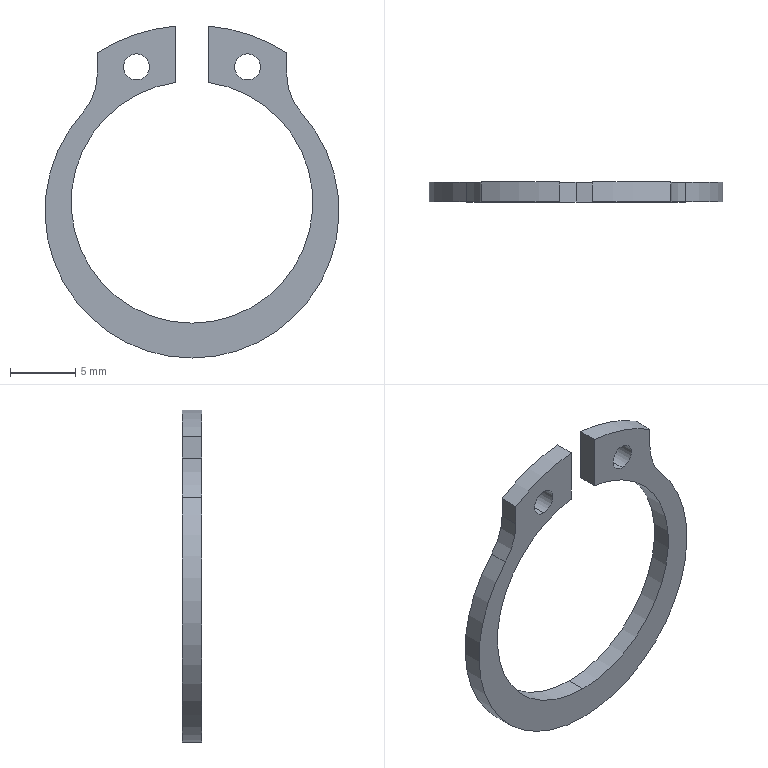Component | SolidWorks | 12-1 | 1 solid | 18 faces | box 22.5 x 1.5 x 25.41 mm | volume 237 mm3 | cylinder 12 | plane 6 | commonest cylinder face diameters 2 x4 18.5 x2 22.5 x2 27.1 x2 9 x2
build123d program:
from build123d import *

# Parameters (mm, degrees)
SKETCH1_R           = 1
BOSS_EXTRUDE1_DEPTH = 1.5
FILLET1_R           = 4.5


with BuildPart() as part:
    # Sketch1 → Boss-Extrude1 (new body)
    with BuildSketch(Plane(origin=(0, 0, 0), x_dir=(1, 0, 0), z_dir=(0, 1, 0))):
        with BuildLine():
            Line((7.25, -11.447), (7.25, -7.932))
            ThreePointArc((7.25, -7.932), (0, 11.92), (-7.25, -7.932))
            Line((-7.25, -7.932), (-7.25, -11.447))
            ThreePointArc((-7.25, -11.447), (-4.371, -12.826), (-1.25, -13.492))
            Line((-1.25, -13.492), (-1.25, -9.165))
            ThreePointArc((-1.25, -9.165), (0, 9.25), (1.25, -9.165))
            Line((1.25, -9.165), (1.25, -13.492))
            ThreePointArc((1.25, -13.492), (4.371, -12.826), (7.25, -11.447))
        make_face()
        with Locations(Location((-4.25, -10.362, 0), (0, 0, 270))):
            Circle(SKETCH1_R, mode=Mode.SUBTRACT)
        with Locations(Location((4.25, -10.362, 0), (0, 0, 90))):
            Circle(SKETCH1_R, mode=Mode.SUBTRACT)
    extrude(amount=BOSS_EXTRUDE1_DEPTH)

    # Fillet1
    fillet1_edges = [part.edges().sort_by_distance(p)[0] for p in [
        (7.25, 0.75, 7.932),
        (-7.25, 0.75, 7.932),
    ]]
    fillet(fillet1_edges, radius=FILLET1_R)


solid = part.part

# Placed as in the assembly
solid = solid.moved(Location((0, -59.437, 0), (0, 0, 0)))
STEP:
#1=COLOUR_RGB('',0.7922,0.8196,0.9333);
#2=FILL_AREA_STYLE_COLOUR('',#1);
#3=FILL_AREA_STYLE('',(#2));
#4=SURFACE_STYLE_FILL_AREA(#3);
#5=SURFACE_SIDE_STYLE('',(#4));
#6=SURFACE_STYLE_USAGE(.BOTH.,#5);
#7=PRESENTATION_STYLE_ASSIGNMENT((#6));
#8=CARTESIAN_POINT('',(0.1673,-2.281,0.3686));
#9=VERTEX_POINT('',#8);
#10=CARTESIAN_POINT('',(0.1673,-2.281,0.4473));
#11=VERTEX_POINT('',#10);
#12=CARTESIAN_POINT('',(0.1673,-2.281,0.408));
#13=DIRECTION('',(0.,1.,0.));
#14=DIRECTION('',(0.,0.,-1.));
#15=AXIS2_PLACEMENT_3D('',#12,#13,#14);
#16=CIRCLE('',#15,0.03937);
#17=EDGE_CURVE('',#9,#11,#16,.T.);
#18=ORIENTED_EDGE('',*,*,#17,.T.);
#19=CARTESIAN_POINT('',(0.1673,-2.34,0.4473));
#20=VERTEX_POINT('',#19);
#21=CARTESIAN_POINT('',(0.1673,-2.281,0.4473));
#22=DIRECTION('',(0.,-1.,0.));
#23=VECTOR('',#22,39.37);
#24=LINE('',#21,#23);
#25=EDGE_CURVE('',#11,#20,#24,.T.);
#26=ORIENTED_EDGE('',*,*,#25,.T.);
#27=CARTESIAN_POINT('',(0.1673,-2.34,0.3686));
#28=VERTEX_POINT('',#27);
#29=CARTESIAN_POINT('',(0.1673,-2.34,0.408));
#30=DIRECTION('',(0.,1.,0.));
#31=DIRECTION('',(0.,0.,-1.));
#32=AXIS2_PLACEMENT_3D('',#29,#30,#31);
#33=CIRCLE('',#32,0.03937);
#34=EDGE_CURVE('',#28,#20,#33,.T.);
#35=ORIENTED_EDGE('',*,*,#34,.F.);
#36=CARTESIAN_POINT('',(0.1673,-2.281,0.3686));
#37=DIRECTION('',(0.,-1.,0.));
#38=VECTOR('',#37,39.37);
#39=LINE('',#36,#38);
#40=EDGE_CURVE('',#9,#28,#39,.T.);
#41=ORIENTED_EDGE('',*,*,#40,.F.);
#42=EDGE_LOOP('',(#18,#26,#35,#41));
#43=FACE_OUTER_BOUND('',#42,.T.);
#44=CARTESIAN_POINT('',(0.1673,-2.281,0.408));
#45=DIRECTION('',(0.,-1.,0.));
#46=DIRECTION('',(0.,0.,-1.));
#47=AXIS2_PLACEMENT_3D('',#44,#45,#46);
#48=CYLINDRICAL_SURFACE('',#47,0.03937);
#49=ADVANCED_FACE('',(#43),#48,.F.);
#50=CARTESIAN_POINT('',(-0.1673,-2.281,0.3686));
#51=VERTEX_POINT('',#50);
#52=CARTESIAN_POINT('',(-0.1673,-2.281,0.4473));
#53=VERTEX_POINT('',#52);
#54=CARTESIAN_POINT('',(-0.1673,-2.281,0.408));
#55=DIRECTION('',(0.,1.,0.));
#56=DIRECTION('',(0.,0.,1.));
#57=AXIS2_PLACEMENT_3D('',#54,#55,#56);
#58=CIRCLE('',#57,0.03937);
#59=EDGE_CURVE('',#51,#53,#58,.T.);
#60=ORIENTED_EDGE('',*,*,#59,.T.);
#61=CARTESIAN_POINT('',(-0.1673,-2.34,0.4473));
#62=VERTEX_POINT('',#61);
#63=CARTESIAN_POINT('',(-0.1673,-2.281,0.4473));
#64=DIRECTION('',(0.,-1.,0.));
#65=VECTOR('',#64,39.37);
#66=LINE('',#63,#65);
#67=EDGE_CURVE('',#53,#62,#66,.T.);
#68=ORIENTED_EDGE('',*,*,#67,.T.);
#69=CARTESIAN_POINT('',(-0.1673,-2.34,0.3686));
#70=VERTEX_POINT('',#69);
#71=CARTESIAN_POINT('',(-0.1673,-2.34,0.408));
#72=DIRECTION('',(0.,1.,0.));
#73=DIRECTION('',(0.,0.,1.));
#74=AXIS2_PLACEMENT_3D('',#71,#72,#73);
#75=CIRCLE('',#74,0.03937);
#76=EDGE_CURVE('',#70,#62,#75,.T.);
#77=ORIENTED_EDGE('',*,*,#76,.F.);
#78=CARTESIAN_POINT('',(-0.1673,-2.281,0.3686));
#79=DIRECTION('',(0.,-1.,0.));
#80=VECTOR('',#79,39.37);
#81=LINE('',#78,#80);
#82=EDGE_CURVE('',#51,#70,#81,.T.);
#83=ORIENTED_EDGE('',*,*,#82,.F.);
#84=EDGE_LOOP('',(#60,#68,#77,#83));
#85=FACE_OUTER_BOUND('',#84,.T.);
#86=CARTESIAN_POINT('',(-0.1673,-2.281,0.408));
#87=DIRECTION('',(0.,-1.,0.));
#88=DIRECTION('',(0.,0.,-1.));
#89=AXIS2_PLACEMENT_3D('',#86,#87,#88);
#90=CYLINDRICAL_SURFACE('',#89,0.03937);
#91=ADVANCED_FACE('',(#85),#90,.F.);
#92=CARTESIAN_POINT('',(0.,-2.281,-0.3642));
#93=VERTEX_POINT('',#92);
#94=CARTESIAN_POINT('',(0.04921,-2.281,0.3608));
#95=VERTEX_POINT('',#94);
#96=CARTESIAN_POINT('',(0.,-2.281,0.));
#97=DIRECTION('',(0.,-1.,0.));
#98=DIRECTION('',(0.,0.,1.));
#99=AXIS2_PLACEMENT_3D('',#96,#97,#98);
#100=CIRCLE('',#99,0.3642);
#101=EDGE_CURVE('',#93,#95,#100,.T.);
#102=ORIENTED_EDGE('',*,*,#101,.F.);
#103=CARTESIAN_POINT('',(0.,-2.34,-0.3642));
#104=VERTEX_POINT('',#103);
#105=CARTESIAN_POINT('',(0.,-2.281,-0.3642));
#106=DIRECTION('',(0.,-1.,0.));
#107=VECTOR('',#106,39.37);
#108=LINE('',#105,#107);
#109=EDGE_CURVE('',#93,#104,#108,.T.);
#110=ORIENTED_EDGE('',*,*,#109,.T.);
#111=CARTESIAN_POINT('',(0.04921,-2.34,0.3608));
#112=VERTEX_POINT('',#111);
#113=CARTESIAN_POINT('',(0.,-2.34,0.));
#114=DIRECTION('',(0.,-1.,0.));
#115=DIRECTION('',(0.,0.,1.));
#116=AXIS2_PLACEMENT_3D('',#113,#114,#115);
#117=CIRCLE('',#116,0.3642);
#118=EDGE_CURVE('',#104,#112,#117,.T.);
#119=ORIENTED_EDGE('',*,*,#118,.T.);
#120=CARTESIAN_POINT('',(0.04921,-2.281,0.3608));
#121=DIRECTION('',(0.,-1.,0.));
#122=VECTOR('',#121,39.37);
#123=LINE('',#120,#122);
#124=EDGE_CURVE('',#95,#112,#123,.T.);
#125=ORIENTED_EDGE('',*,*,#124,.F.);
#126=EDGE_LOOP('',(#102,#110,#119,#125));
#127=FACE_OUTER_BOUND('',#126,.T.);
#128=CARTESIAN_POINT('',(0.,-2.281,0.));
#129=DIRECTION('',(0.,-1.,0.));
#130=DIRECTION('',(0.,0.,-1.));
#131=AXIS2_PLACEMENT_3D('',#128,#129,#130);
#132=CYLINDRICAL_SURFACE('',#131,0.3642);
#133=ADVANCED_FACE('',(#127),#132,.F.);
#134=CARTESIAN_POINT('',(0.,-2.281,-0.4693));
#135=VERTEX_POINT('',#134);
#136=CARTESIAN_POINT('',(-0.3304,-2.281,0.2686));
#137=VERTEX_POINT('',#136);
#138=CARTESIAN_POINT('',(0.,-2.281,-0.02638));
#139=DIRECTION('',(0.,1.,0.));
#140=DIRECTION('',(0.,0.,1.));
#141=AXIS2_PLACEMENT_3D('',#138,#139,#140);
#142=CIRCLE('',#141,0.4429);
#143=EDGE_CURVE('',#135,#137,#142,.T.);
#144=ORIENTED_EDGE('',*,*,#143,.F.);
#145=CARTESIAN_POINT('',(0.,-2.34,-0.4693));
#146=VERTEX_POINT('',#145);
#147=CARTESIAN_POINT('',(0.,-2.281,-0.4693));
#148=DIRECTION('',(0.,-1.,0.));
#149=VECTOR('',#148,39.37);
#150=LINE('',#147,#149);
#151=EDGE_CURVE('',#135,#146,#150,.T.);
#152=ORIENTED_EDGE('',*,*,#151,.T.);
#153=CARTESIAN_POINT('',(-0.3304,-2.34,0.2686));
#154=VERTEX_POINT('',#153);
#155=CARTESIAN_POINT('',(0.,-2.34,-0.02638));
#156=DIRECTION('',(0.,1.,0.));
#157=DIRECTION('',(0.,0.,1.));
#158=AXIS2_PLACEMENT_3D('',#155,#156,#157);
#159=CIRCLE('',#158,0.4429);
#160=EDGE_CURVE('',#146,#154,#159,.T.);
#161=ORIENTED_EDGE('',*,*,#160,.T.);
#162=CARTESIAN_POINT('',(-0.3304,-2.281,0.2686));
#163=DIRECTION('',(0.,1.,0.));
#164=VECTOR('',#163,39.37);
#165=LINE('',#162,#164);
#166=EDGE_CURVE('',#154,#137,#165,.T.);
#167=ORIENTED_EDGE('',*,*,#166,.T.);
#168=EDGE_LOOP('',(#144,#152,#161,#167));
#169=FACE_OUTER_BOUND('',#168,.T.);
#170=CARTESIAN_POINT('',(0.,-2.281,-0.02638));
#171=DIRECTION('',(0.,-1.,0.));
#172=DIRECTION('',(0.,0.,-1.));
#173=AXIS2_PLACEMENT_3D('',#170,#171,#172);
#174=CYLINDRICAL_SURFACE('',#173,0.4429);
#175=ADVANCED_FACE('',(#169),#174,.T.);
#176=ORIENTED_EDGE('',*,*,#59,.F.);
#177=CARTESIAN_POINT('',(-0.1673,-2.281,0.408));
#178=DIRECTION('',(0.,1.,0.));
#179=DIRECTION('',(0.,0.,1.));
#180=AXIS2_PLACEMENT_3D('',#177,#178,#179);
#181=CIRCLE('',#180,0.03937);
#182=EDGE_CURVE('',#53,#51,#181,.T.);
#183=ORIENTED_EDGE('',*,*,#182,.F.);
#184=EDGE_LOOP('',(#176,#183));
#185=FACE_BOUND('',#184,.T.);
#186=CARTESIAN_POINT('',(0.2854,-2.281,0.4507));
#187=VERTEX_POINT('',#186);
#188=CARTESIAN_POINT('',(0.2854,-2.281,0.3865));
#189=VERTEX_POINT('',#188);
#190=CARTESIAN_POINT('',(0.2854,-2.281,0.4507));
#191=DIRECTION('',(0.,0.,-1.));
#192=VECTOR('',#191,39.37);
#193=LINE('',#190,#192);
#194=EDGE_CURVE('',#187,#189,#193,.T.);
#195=ORIENTED_EDGE('',*,*,#194,.T.);
#196=CARTESIAN_POINT('',(0.3304,-2.281,0.2686));
#197=VERTEX_POINT('',#196);
#198=CARTESIAN_POINT('',(0.4626,-2.281,0.3865));
#199=DIRECTION('',(0.,-1.,0.));
#200=DIRECTION('',(-0.,0.,1.));
#201=AXIS2_PLACEMENT_3D('',#198,#199,#200);
#202=CIRCLE('',#201,0.1772);
#203=EDGE_CURVE('',#189,#197,#202,.T.);
#204=ORIENTED_EDGE('',*,*,#203,.T.);
#205=CARTESIAN_POINT('',(0.,-2.281,-0.02638));
#206=DIRECTION('',(0.,1.,0.));
#207=DIRECTION('',(0.,0.,1.));
#208=AXIS2_PLACEMENT_3D('',#205,#206,#207);
#209=CIRCLE('',#208,0.4429);
#210=EDGE_CURVE('',#197,#135,#209,.T.);
#211=ORIENTED_EDGE('',*,*,#210,.T.);
#212=ORIENTED_EDGE('',*,*,#143,.T.);
#213=CARTESIAN_POINT('',(-0.2854,-2.281,0.3865));
#214=VERTEX_POINT('',#213);
#215=CARTESIAN_POINT('',(-0.4626,-2.281,0.3865));
#216=DIRECTION('',(0.,-1.,0.));
#217=DIRECTION('',(0.,0.,1.));
#218=AXIS2_PLACEMENT_3D('',#215,#216,#217);
#219=CIRCLE('',#218,0.1772);
#220=EDGE_CURVE('',#137,#214,#219,.T.);
#221=ORIENTED_EDGE('',*,*,#220,.T.);
#222=CARTESIAN_POINT('',(-0.2854,-2.281,0.4507));
#223=VERTEX_POINT('',#222);
#224=CARTESIAN_POINT('',(-0.2854,-2.281,0.4507));
#225=DIRECTION('',(0.,0.,1.));
#226=VECTOR('',#225,39.37);
#227=LINE('',#224,#226);
#228=EDGE_CURVE('',#214,#223,#227,.T.);
#229=ORIENTED_EDGE('',*,*,#228,.T.);
#230=CARTESIAN_POINT('',(-0.04921,-2.281,0.5312));
#231=VERTEX_POINT('',#230);
#232=CARTESIAN_POINT('',(0.,-2.281,0.));
#233=DIRECTION('',(0.,1.,0.));
#234=DIRECTION('',(0.,0.,1.));
#235=AXIS2_PLACEMENT_3D('',#232,#233,#234);
#236=CIRCLE('',#235,0.5335);
#237=EDGE_CURVE('',#223,#231,#236,.T.);
#238=ORIENTED_EDGE('',*,*,#237,.T.);
#239=CARTESIAN_POINT('',(-0.04921,-2.281,0.3608));
#240=VERTEX_POINT('',#239);
#241=CARTESIAN_POINT('',(-0.04921,-2.281,0.3608));
#242=DIRECTION('',(-0.,0.,-1.));
#243=VECTOR('',#242,39.37);
#244=LINE('',#241,#243);
#245=EDGE_CURVE('',#231,#240,#244,.T.);
#246=ORIENTED_EDGE('',*,*,#245,.T.);
#247=CARTESIAN_POINT('',(0.,-2.281,0.));
#248=DIRECTION('',(0.,-1.,0.));
#249=DIRECTION('',(0.,0.,1.));
#250=AXIS2_PLACEMENT_3D('',#247,#248,#249);
#251=CIRCLE('',#250,0.3642);
#252=EDGE_CURVE('',#240,#93,#251,.T.);
#253=ORIENTED_EDGE('',*,*,#252,.T.);
#254=ORIENTED_EDGE('',*,*,#101,.T.);
#255=CARTESIAN_POINT('',(0.04921,-2.281,0.5312));
#256=VERTEX_POINT('',#255);
#257=CARTESIAN_POINT('',(0.04921,-2.281,0.3608));
#258=DIRECTION('',(-0.,0.,1.));
#259=VECTOR('',#258,39.37);
#260=LINE('',#257,#259);
#261=EDGE_CURVE('',#95,#256,#260,.T.);
#262=ORIENTED_EDGE('',*,*,#261,.T.);
#263=CARTESIAN_POINT('',(0.,-2.281,0.));
#264=DIRECTION('',(0.,1.,0.));
#265=DIRECTION('',(0.,0.,1.));
#266=AXIS2_PLACEMENT_3D('',#263,#264,#265);
#267=CIRCLE('',#266,0.5335);
#268=EDGE_CURVE('',#256,#187,#267,.T.);
#269=ORIENTED_EDGE('',*,*,#268,.T.);
#270=EDGE_LOOP('',(#195,#204,#211,#212,#221,#229,#238,#246,#253,#254,#262,#269));
#271=FACE_OUTER_BOUND('',#270,.T.);
#272=ORIENTED_EDGE('',*,*,#17,.F.);
#273=CARTESIAN_POINT('',(0.1673,-2.281,0.408));
#274=DIRECTION('',(0.,1.,0.));
#275=DIRECTION('',(0.,0.,-1.));
#276=AXIS2_PLACEMENT_3D('',#273,#274,#275);
#277=CIRCLE('',#276,0.03937);
#278=EDGE_CURVE('',#11,#9,#277,.T.);
#279=ORIENTED_EDGE('',*,*,#278,.F.);
#280=EDGE_LOOP('',(#272,#279));
#281=FACE_BOUND('',#280,.T.);
#282=CARTESIAN_POINT('',(0.,-2.281,-0.02638));
#283=DIRECTION('',(0.,1.,0.));
#284=DIRECTION('',(0.,0.,1.));
#285=AXIS2_PLACEMENT_3D('',#282,#283,#284);
#286=PLANE('',#285);
#287=ADVANCED_FACE('',(#185,#271,#281),#286,.T.);
#288=CARTESIAN_POINT('',(0.3304,-2.34,0.2686));
#289=VERTEX_POINT('',#288);
#290=CARTESIAN_POINT('',(0.,-2.34,-0.02638));
#291=DIRECTION('',(0.,1.,0.));
#292=DIRECTION('',(0.,0.,1.));
#293=AXIS2_PLACEMENT_3D('',#290,#291,#292);
#294=CIRCLE('',#293,0.4429);
#295=EDGE_CURVE('',#289,#146,#294,.T.);
#296=ORIENTED_EDGE('',*,*,#295,.F.);
#297=CARTESIAN_POINT('',(0.2854,-2.34,0.3865));
#298=VERTEX_POINT('',#297);
#299=CARTESIAN_POINT('',(0.4626,-2.34,0.3865));
#300=DIRECTION('',(0.,1.,0.));
#301=DIRECTION('',(0.,0.,1.));
#302=AXIS2_PLACEMENT_3D('',#299,#300,#301);
#303=CIRCLE('',#302,0.1772);
#304=EDGE_CURVE('',#289,#298,#303,.T.);
#305=ORIENTED_EDGE('',*,*,#304,.T.);
#306=CARTESIAN_POINT('',(0.2854,-2.34,0.4507));
#307=VERTEX_POINT('',#306);
#308=CARTESIAN_POINT('',(0.2854,-2.34,0.4507));
#309=DIRECTION('',(0.,0.,-1.));
#310=VECTOR('',#309,39.37);
#311=LINE('',#308,#310);
#312=EDGE_CURVE('',#307,#298,#311,.T.);
#313=ORIENTED_EDGE('',*,*,#312,.F.);
#314=CARTESIAN_POINT('',(0.04921,-2.34,0.5312));
#315=VERTEX_POINT('',#314);
#316=CARTESIAN_POINT('',(0.,-2.34,0.));
#317=DIRECTION('',(0.,1.,0.));
#318=DIRECTION('',(0.,0.,1.));
#319=AXIS2_PLACEMENT_3D('',#316,#317,#318);
#320=CIRCLE('',#319,0.5335);
#321=EDGE_CURVE('',#315,#307,#320,.T.);
#322=ORIENTED_EDGE('',*,*,#321,.F.);
#323=CARTESIAN_POINT('',(0.04921,-2.34,0.3608));
#324=DIRECTION('',(-0.,0.,1.));
#325=VECTOR('',#324,39.37);
#326=LINE('',#323,#325);
#327=EDGE_CURVE('',#112,#315,#326,.T.);
#328=ORIENTED_EDGE('',*,*,#327,.F.);
#329=ORIENTED_EDGE('',*,*,#118,.F.);
#330=CARTESIAN_POINT('',(-0.04921,-2.34,0.3608));
#331=VERTEX_POINT('',#330);
#332=CARTESIAN_POINT('',(0.,-2.34,0.));
#333=DIRECTION('',(0.,-1.,0.));
#334=DIRECTION('',(0.,0.,1.));
#335=AXIS2_PLACEMENT_3D('',#332,#333,#334);
#336=CIRCLE('',#335,0.3642);
#337=EDGE_CURVE('',#331,#104,#336,.T.);
#338=ORIENTED_EDGE('',*,*,#337,.F.);
#339=CARTESIAN_POINT('',(-0.04921,-2.34,0.5312));
#340=VERTEX_POINT('',#339);
#341=CARTESIAN_POINT('',(-0.04921,-2.34,0.3608));
#342=DIRECTION('',(-0.,0.,-1.));
#343=VECTOR('',#342,39.37);
#344=LINE('',#341,#343);
#345=EDGE_CURVE('',#340,#331,#344,.T.);
#346=ORIENTED_EDGE('',*,*,#345,.F.);
#347=CARTESIAN_POINT('',(-0.2854,-2.34,0.4507));
#348=VERTEX_POINT('',#347);
#349=CARTESIAN_POINT('',(0.,-2.34,0.));
#350=DIRECTION('',(0.,1.,0.));
#351=DIRECTION('',(0.,0.,1.));
#352=AXIS2_PLACEMENT_3D('',#349,#350,#351);
#353=CIRCLE('',#352,0.5335);
#354=EDGE_CURVE('',#348,#340,#353,.T.);
#355=ORIENTED_EDGE('',*,*,#354,.F.);
#356=CARTESIAN_POINT('',(-0.2854,-2.34,0.3865));
#357=VERTEX_POINT('',#356);
#358=CARTESIAN_POINT('',(-0.2854,-2.34,0.4507));
#359=DIRECTION('',(0.,0.,1.));
#360=VECTOR('',#359,39.37);
#361=LINE('',#358,#360);
#362=EDGE_CURVE('',#357,#348,#361,.T.);
#363=ORIENTED_EDGE('',*,*,#362,.F.);
#364=CARTESIAN_POINT('',(-0.4626,-2.34,0.3865));
#365=DIRECTION('',(0.,1.,0.));
#366=DIRECTION('',(0.,0.,1.));
#367=AXIS2_PLACEMENT_3D('',#364,#365,#366);
#368=CIRCLE('',#367,0.1772);
#369=EDGE_CURVE('',#357,#154,#368,.T.);
#370=ORIENTED_EDGE('',*,*,#369,.T.);
#371=ORIENTED_EDGE('',*,*,#160,.F.);
#372=EDGE_LOOP('',(#296,#305,#313,#322,#328,#329,#338,#346,#355,#363,#370,#371));
#373=FACE_OUTER_BOUND('',#372,.T.);
#374=ORIENTED_EDGE('',*,*,#76,.T.);
#375=CARTESIAN_POINT('',(-0.1673,-2.34,0.408));
#376=DIRECTION('',(0.,1.,0.));
#377=DIRECTION('',(0.,0.,1.));
#378=AXIS2_PLACEMENT_3D('',#375,#376,#377);
#379=CIRCLE('',#378,0.03937);
#380=EDGE_CURVE('',#62,#70,#379,.T.);
#381=ORIENTED_EDGE('',*,*,#380,.T.);
#382=EDGE_LOOP('',(#374,#381));
#383=FACE_BOUND('',#382,.T.);
#384=ORIENTED_EDGE('',*,*,#34,.T.);
#385=CARTESIAN_POINT('',(0.1673,-2.34,0.408));
#386=DIRECTION('',(0.,1.,0.));
#387=DIRECTION('',(0.,0.,-1.));
#388=AXIS2_PLACEMENT_3D('',#385,#386,#387);
#389=CIRCLE('',#388,0.03937);
#390=EDGE_CURVE('',#20,#28,#389,.T.);
#391=ORIENTED_EDGE('',*,*,#390,.T.);
#392=EDGE_LOOP('',(#384,#391));
#393=FACE_BOUND('',#392,.T.);
#394=CARTESIAN_POINT('',(0.,-2.34,-0.02638));
#395=DIRECTION('',(0.,1.,0.));
#396=DIRECTION('',(0.,0.,1.));
#397=AXIS2_PLACEMENT_3D('',#394,#395,#396);
#398=PLANE('',#397);
#399=ADVANCED_FACE('',(#373,#383,#393),#398,.F.);
#400=ORIENTED_EDGE('',*,*,#151,.F.);
#401=ORIENTED_EDGE('',*,*,#210,.F.);
#402=CARTESIAN_POINT('',(0.3304,-2.281,0.2686));
#403=DIRECTION('',(0.,-1.,0.));
#404=VECTOR('',#403,39.37);
#405=LINE('',#402,#404);
#406=EDGE_CURVE('',#197,#289,#405,.T.);
#407=ORIENTED_EDGE('',*,*,#406,.T.);
#408=ORIENTED_EDGE('',*,*,#295,.T.);
#409=EDGE_LOOP('',(#400,#401,#407,#408));
#410=FACE_OUTER_BOUND('',#409,.T.);
#411=CARTESIAN_POINT('',(0.,-2.281,-0.02638));
#412=DIRECTION('',(0.,-1.,0.));
#413=DIRECTION('',(0.,0.,-1.));
#414=AXIS2_PLACEMENT_3D('',#411,#412,#413);
#415=CYLINDRICAL_SURFACE('',#414,0.4429);
#416=ADVANCED_FACE('',(#410),#415,.T.);
#417=ORIENTED_EDGE('',*,*,#228,.F.);
#418=CARTESIAN_POINT('',(-0.2854,-2.34,0.3865));
#419=DIRECTION('',(0.,-1.,0.));
#420=VECTOR('',#419,39.37);
#421=LINE('',#418,#420);
#422=EDGE_CURVE('',#214,#357,#421,.T.);
#423=ORIENTED_EDGE('',*,*,#422,.T.);
#424=ORIENTED_EDGE('',*,*,#362,.T.);
#425=CARTESIAN_POINT('',(-0.2854,-2.281,0.4507));
#426=DIRECTION('',(0.,-1.,0.));
#427=VECTOR('',#426,39.37);
#428=LINE('',#425,#427);
#429=EDGE_CURVE('',#223,#348,#428,.T.);
#430=ORIENTED_EDGE('',*,*,#429,.F.);
#431=EDGE_LOOP('',(#417,#423,#424,#430));
#432=FACE_OUTER_BOUND('',#431,.T.);
#433=CARTESIAN_POINT('',(-0.2854,-2.281,0.4507));
#434=DIRECTION('',(1.,0.,0.));
#435=DIRECTION('',(0.,0.,-1.));
#436=AXIS2_PLACEMENT_3D('',#433,#434,#435);
#437=PLANE('',#436);
#438=ADVANCED_FACE('',(#432),#437,.F.);
#439=ORIENTED_EDGE('',*,*,#354,.T.);
#440=CARTESIAN_POINT('',(-0.04921,-2.281,0.5312));
#441=DIRECTION('',(0.,-1.,0.));
#442=VECTOR('',#441,39.37);
#443=LINE('',#440,#442);
#444=EDGE_CURVE('',#231,#340,#443,.T.);
#445=ORIENTED_EDGE('',*,*,#444,.F.);
#446=ORIENTED_EDGE('',*,*,#237,.F.);
#447=ORIENTED_EDGE('',*,*,#429,.T.);
#448=EDGE_LOOP('',(#439,#445,#446,#447));
#449=FACE_OUTER_BOUND('',#448,.T.);
#450=CARTESIAN_POINT('',(0.,-2.281,0.));
#451=DIRECTION('',(0.,-1.,0.));
#452=DIRECTION('',(0.,0.,-1.));
#453=AXIS2_PLACEMENT_3D('',#450,#451,#452);
#454=CYLINDRICAL_SURFACE('',#453,0.5335);
#455=ADVANCED_FACE('',(#449),#454,.T.);
#456=ORIENTED_EDGE('',*,*,#345,.T.);
#457=CARTESIAN_POINT('',(-0.04921,-2.281,0.3608));
#458=DIRECTION('',(0.,-1.,0.));
#459=VECTOR('',#458,39.37);
#460=LINE('',#457,#459);
#461=EDGE_CURVE('',#240,#331,#460,.T.);
#462=ORIENTED_EDGE('',*,*,#461,.F.);
#463=ORIENTED_EDGE('',*,*,#245,.F.);
#464=ORIENTED_EDGE('',*,*,#444,.T.);
#465=EDGE_LOOP('',(#456,#462,#463,#464));
#466=FACE_OUTER_BOUND('',#465,.T.);
#467=CARTESIAN_POINT('',(-0.04921,-2.281,0.3608));
#468=DIRECTION('',(-1.,0.,0.));
#469=DIRECTION('',(0.,0.,1.));
#470=AXIS2_PLACEMENT_3D('',#467,#468,#469);
#471=PLANE('',#470);
#472=ADVANCED_FACE('',(#466),#471,.F.);
#473=ORIENTED_EDGE('',*,*,#109,.F.);
#474=ORIENTED_EDGE('',*,*,#252,.F.);
#475=ORIENTED_EDGE('',*,*,#461,.T.);
#476=ORIENTED_EDGE('',*,*,#337,.T.);
#477=EDGE_LOOP('',(#473,#474,#475,#476));
#478=FACE_OUTER_BOUND('',#477,.T.);
#479=CARTESIAN_POINT('',(0.,-2.281,0.));
#480=DIRECTION('',(0.,-1.,0.));
#481=DIRECTION('',(0.,0.,-1.));
#482=AXIS2_PLACEMENT_3D('',#479,#480,#481);
#483=CYLINDRICAL_SURFACE('',#482,0.3642);
#484=ADVANCED_FACE('',(#478),#483,.F.);
#485=ORIENTED_EDGE('',*,*,#327,.T.);
#486=CARTESIAN_POINT('',(0.04921,-2.281,0.5312));
#487=DIRECTION('',(0.,-1.,0.));
#488=VECTOR('',#487,39.37);
#489=LINE('',#486,#488);
#490=EDGE_CURVE('',#256,#315,#489,.T.);
#491=ORIENTED_EDGE('',*,*,#490,.F.);
#492=ORIENTED_EDGE('',*,*,#261,.F.);
#493=ORIENTED_EDGE('',*,*,#124,.T.);
#494=EDGE_LOOP('',(#485,#491,#492,#493));
#495=FACE_OUTER_BOUND('',#494,.T.);
#496=CARTESIAN_POINT('',(0.04921,-2.281,0.3608));
#497=DIRECTION('',(1.,0.,0.));
#498=DIRECTION('',(0.,0.,-1.));
#499=AXIS2_PLACEMENT_3D('',#496,#497,#498);
#500=PLANE('',#499);
#501=ADVANCED_FACE('',(#495),#500,.F.);
#502=ORIENTED_EDGE('',*,*,#321,.T.);
#503=CARTESIAN_POINT('',(0.2854,-2.281,0.4507));
#504=DIRECTION('',(0.,-1.,0.));
#505=VECTOR('',#504,39.37);
#506=LINE('',#503,#505);
#507=EDGE_CURVE('',#187,#307,#506,.T.);
#508=ORIENTED_EDGE('',*,*,#507,.F.);
#509=ORIENTED_EDGE('',*,*,#268,.F.);
#510=ORIENTED_EDGE('',*,*,#490,.T.);
#511=EDGE_LOOP('',(#502,#508,#509,#510));
#512=FACE_OUTER_BOUND('',#511,.T.);
#513=CARTESIAN_POINT('',(0.,-2.281,0.));
#514=DIRECTION('',(0.,-1.,0.));
#515=DIRECTION('',(0.,0.,-1.));
#516=AXIS2_PLACEMENT_3D('',#513,#514,#515);
#517=CYLINDRICAL_SURFACE('',#516,0.5335);
#518=ADVANCED_FACE('',(#512),#517,.T.);
#519=ORIENTED_EDGE('',*,*,#312,.T.);
#520=CARTESIAN_POINT('',(0.2854,-2.281,0.3865));
#521=DIRECTION('',(0.,1.,0.));
#522=VECTOR('',#521,39.37);
#523=LINE('',#520,#522);
#524=EDGE_CURVE('',#298,#189,#523,.T.);
#525=ORIENTED_EDGE('',*,*,#524,.T.);
#526=ORIENTED_EDGE('',*,*,#194,.F.);
#527=ORIENTED_EDGE('',*,*,#507,.T.);
#528=EDGE_LOOP('',(#519,#525,#526,#527));
#529=FACE_OUTER_BOUND('',#528,.T.);
#530=CARTESIAN_POINT('',(0.2854,-2.281,0.4507));
#531=DIRECTION('',(-1.,0.,0.));
#532=DIRECTION('',(0.,0.,1.));
#533=AXIS2_PLACEMENT_3D('',#530,#531,#532);
#534=PLANE('',#533);
#535=ADVANCED_FACE('',(#529),#534,.F.);
#536=ORIENTED_EDGE('',*,*,#67,.F.);
#537=ORIENTED_EDGE('',*,*,#182,.T.);
#538=ORIENTED_EDGE('',*,*,#82,.T.);
#539=ORIENTED_EDGE('',*,*,#380,.F.);
#540=EDGE_LOOP('',(#536,#537,#538,#539));
#541=FACE_OUTER_BOUND('',#540,.T.);
#542=CARTESIAN_POINT('',(-0.1673,-2.281,0.408));
#543=DIRECTION('',(0.,-1.,0.));
#544=DIRECTION('',(0.,0.,-1.));
#545=AXIS2_PLACEMENT_3D('',#542,#543,#544);
#546=CYLINDRICAL_SURFACE('',#545,0.03937);
#547=ADVANCED_FACE('',(#541),#546,.F.);
#548=ORIENTED_EDGE('',*,*,#25,.F.);
#549=ORIENTED_EDGE('',*,*,#278,.T.);
#550=ORIENTED_EDGE('',*,*,#40,.T.);
#551=ORIENTED_EDGE('',*,*,#390,.F.);
#552=EDGE_LOOP('',(#548,#549,#550,#551));
#553=FACE_OUTER_BOUND('',#552,.T.);
#554=CARTESIAN_POINT('',(0.1673,-2.281,0.408));
#555=DIRECTION('',(0.,-1.,0.));
#556=DIRECTION('',(0.,0.,-1.));
#557=AXIS2_PLACEMENT_3D('',#554,#555,#556);
#558=CYLINDRICAL_SURFACE('',#557,0.03937);
#559=ADVANCED_FACE('',(#553),#558,.F.);
#560=ORIENTED_EDGE('',*,*,#220,.F.);
#561=ORIENTED_EDGE('',*,*,#166,.F.);
#562=ORIENTED_EDGE('',*,*,#369,.F.);
#563=ORIENTED_EDGE('',*,*,#422,.F.);
#564=EDGE_LOOP('',(#560,#561,#562,#563));
#565=FACE_OUTER_BOUND('',#564,.T.);
#566=CARTESIAN_POINT('',(-0.4626,-2.281,0.3865));
#567=DIRECTION('',(0.,-1.,0.));
#568=DIRECTION('',(0.,0.,-1.));
#569=AXIS2_PLACEMENT_3D('',#566,#567,#568);
#570=CYLINDRICAL_SURFACE('',#569,0.1772);
#571=ADVANCED_FACE('',(#565),#570,.F.);
#572=ORIENTED_EDGE('',*,*,#203,.F.);
#573=ORIENTED_EDGE('',*,*,#524,.F.);
#574=ORIENTED_EDGE('',*,*,#304,.F.);
#575=ORIENTED_EDGE('',*,*,#406,.F.);
#576=EDGE_LOOP('',(#572,#573,#574,#575));
#577=FACE_OUTER_BOUND('',#576,.T.);
#578=CARTESIAN_POINT('',(0.4626,-2.281,0.3865));
#579=DIRECTION('',(0.,-1.,0.));
#580=DIRECTION('',(0.,0.,-1.));
#581=AXIS2_PLACEMENT_3D('',#578,#579,#580);
#582=CYLINDRICAL_SURFACE('',#581,0.1772);
#583=ADVANCED_FACE('',(#577),#582,.F.);
#584=CLOSED_SHELL('',(#49,#91,#133,#175,#287,#399,#416,#438,#455,#472,#484,#501,#518,#535,#547,#559,#571,#583));
#585=MANIFOLD_SOLID_BREP('',#584);
#586=STYLED_ITEM('',(#7),#585);
#587=(LENGTH_UNIT()NAMED_UNIT(*)SI_UNIT($,.METRE.));
#588=LENGTH_MEASURE_WITH_UNIT(LENGTH_MEASURE(0.0254),#587);
#589=DIMENSIONAL_EXPONENTS(1.,0.,0.,0.,0.,0.,0.);
#590=(CONVERSION_BASED_UNIT('',#588)LENGTH_UNIT()NAMED_UNIT(#589));
#591=UNCERTAINTY_MEASURE_WITH_UNIT(LENGTH_MEASURE(0.00001),#590,'','');
#592=(NAMED_UNIT(*)PLANE_ANGLE_UNIT()SI_UNIT($,.RADIAN.));
#593=(NAMED_UNIT(*)SI_UNIT($,.STERADIAN.)SOLID_ANGLE_UNIT());
#594=(GEOMETRIC_REPRESENTATION_CONTEXT(3)GLOBAL_UNCERTAINTY_ASSIGNED_CONTEXT((#591))GLOBAL_UNIT_ASSIGNED_CONTEXT((#590,#592,#593))REPRESENTATION_CONTEXT('',''));
#595=MECHANICAL_DESIGN_GEOMETRIC_PRESENTATION_REPRESENTATION('',(#586),#594);
#596=PRESENTATION_LAYER_ASSIGNMENT('','',(#586));
#597=CARTESIAN_POINT('',(0.,0.,0.));
#598=DIRECTION('',(0.,0.,1.));
#599=DIRECTION('',(1.,0.,0.));
#600=AXIS2_PLACEMENT_3D('',#597,#598,#599);
#601=(LENGTH_UNIT()NAMED_UNIT(*)SI_UNIT($,.METRE.));
#602=LENGTH_MEASURE_WITH_UNIT(LENGTH_MEASURE(0.0254),#601);
#603=DIMENSIONAL_EXPONENTS(1.,0.,0.,0.,0.,0.,0.);
#604=(CONVERSION_BASED_UNIT('',#602)LENGTH_UNIT()NAMED_UNIT(#603));
#605=UNCERTAINTY_MEASURE_WITH_UNIT(LENGTH_MEASURE(0.00001),#604,'','');
#606=(NAMED_UNIT(*)PLANE_ANGLE_UNIT()SI_UNIT($,.RADIAN.));
#607=(NAMED_UNIT(*)SI_UNIT($,.STERADIAN.)SOLID_ANGLE_UNIT());
#608=(GEOMETRIC_REPRESENTATION_CONTEXT(3)GLOBAL_UNCERTAINTY_ASSIGNED_CONTEXT((#605))GLOBAL_UNIT_ASSIGNED_CONTEXT((#604,#606,#607))REPRESENTATION_CONTEXT('',''));
#609=ADVANCED_BREP_SHAPE_REPRESENTATION('',(#585,#600),#608);